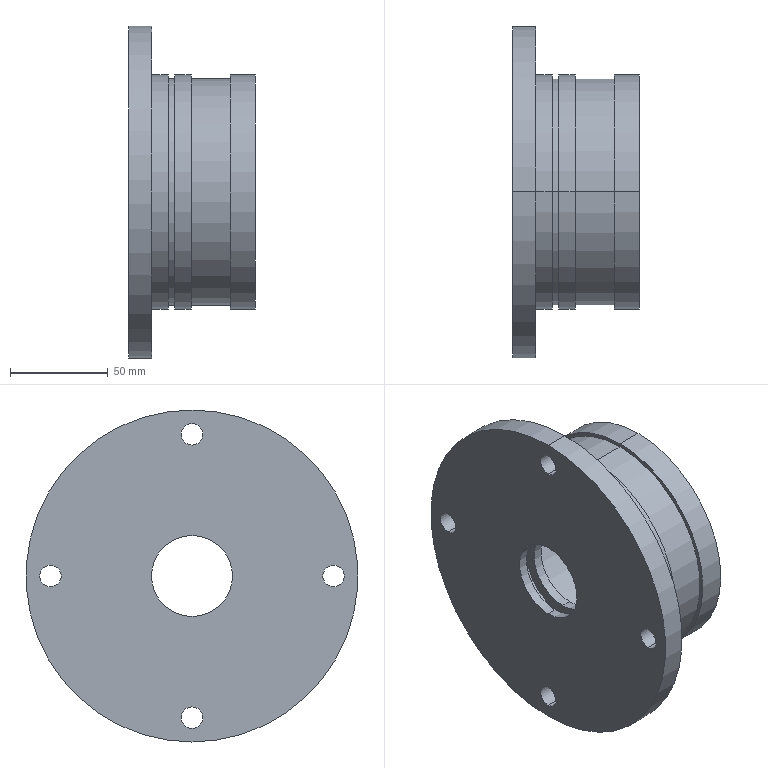Component | SolidWorks | 3FrontCover-1 | 1 solid | 44 faces | box 65 x 170 x 170 mm | volume 391032 mm3 | cylinder 32 | plane 12 | commonest cylinder face diameters 11 x8 120 x6 41.5 x4 116 x4 53 x2 70 x2 100 x2 104 x2
build123d program:
from build123d import *

# Parameters (mm, degrees)
SKETCH74_R           = 85
BOSS_EXTRUDE21_DEPTH = 12
SKETCH75_R           = 60
BOSS_EXTRUDE22_DEPTH = 53
CUT_EXTRUDE18_START  = -33
SKETCH76_2_R         = 60
SKETCH76_2_R_2       = 58
CUT_EXTRUDE18_DEPTH  = 20
CUT_EXTRUDE19_START  = -44.775
SKETCH76_2_2_R       = 60
SKETCH76_2_2_R_2     = 58
CUT_EXTRUDE19_DEPTH  = 3.55
BOSS_EXTRUDE23_START = -8
SKETCH80_R           = 35
BOSS_EXTRUDE23_DEPTH = 15.4
SKETCH81_R           = 20.75
CUT_EXTRUDE20_DEPTH  = 5
SKETCH82_R           = 26.5
CUT_EXTRUDE21_DEPTH  = 5.4
SKETCH83_R           = 20.75
CUT_EXTRUDE22_DEPTH  = 5.4
SKETCH84_R           = 5.5
CUT_EXTRUDE23_DEPTH  = 132.374
CIRPATTERN4_COUNT    = 4


with BuildPart() as part:
    # Sketch74 → Boss-Extrude21 (new body)
    with BuildSketch(Plane(origin=(0, 0, 0), x_dir=(0, 0, -1), z_dir=(1, 0, 0))):
        Circle(SKETCH74_R)
    extrude(amount=BOSS_EXTRUDE21_DEPTH)

    # Sketch75 → Boss-Extrude22 (add)
    with BuildSketch(Plane(origin=(12, 0, 0), x_dir=(0, 0, -1), z_dir=(1, 0, 0))):
        Circle(SKETCH75_R)
    extrude(amount=BOSS_EXTRUDE22_DEPTH)

    # Sketch76_2 → Cut-Extrude18 (cut)
    with BuildSketch(Plane(origin=(65, 0, 0), x_dir=(0, 0, -1), z_dir=(1, 0, 0)).offset(CUT_EXTRUDE18_START)):
        Circle(SKETCH76_2_R)
        Circle(SKETCH76_2_R_2, mode=Mode.SUBTRACT)
    extrude(amount=CUT_EXTRUDE18_DEPTH, mode=Mode.SUBTRACT)

    # Sketch76_2 2 → Cut-Extrude19 (cut)
    with BuildSketch(Plane(origin=(65, 0, 0), x_dir=(0, 0, -1), z_dir=(1, 0, 0)).offset(CUT_EXTRUDE19_START)):
        Circle(SKETCH76_2_2_R)
        Circle(SKETCH76_2_2_R_2, mode=Mode.SUBTRACT)
    extrude(amount=CUT_EXTRUDE19_DEPTH, mode=Mode.SUBTRACT)

    # Sketch78 → Cut-Revolve1 (revolve, cut)
    with BuildSketch(Plane.XY, mode=Mode.PRIVATE) as cut_revolve1_sk:
        Polygon((65, 50), (30, 50), (30, 52), (8, 52), (8, 0), (65, 0), align=None)
    revolve(cut_revolve1_sk.sketch.rotate(Axis((-72.213, 0, 0), (1, 0, 0)), 90), axis=Axis((-72.213, 0, 0), (1, 0, 0)), mode=Mode.SUBTRACT)

    # Sketch80 → Boss-Extrude23 (add)
    with BuildSketch(Plane(origin=(8, 0, 0), x_dir=(0, 0, -1), z_dir=(1, 0, 0)).offset(BOSS_EXTRUDE23_START)):
        with Locations(Location((0, 0, 0), (0, 0, 180))):
            Circle(SKETCH80_R)
    extrude(amount=BOSS_EXTRUDE23_DEPTH)

    # Sketch81 → Cut-Extrude20 (cut)
    with BuildSketch(Plane(origin=(15.4, 0, 0), x_dir=(0, 0, -1), z_dir=(1, 0, 0))):
        Circle(SKETCH81_R)
    extrude(amount=-CUT_EXTRUDE20_DEPTH, mode=Mode.SUBTRACT)

    # Sketch82 → Cut-Extrude21 (cut)
    with BuildSketch(Plane(origin=(10.4, 0, 0), x_dir=(0, 0, -1), z_dir=(1, 0, 0))):
        Circle(SKETCH82_R)
    extrude(amount=-CUT_EXTRUDE21_DEPTH, mode=Mode.SUBTRACT)

    # Sketch83 → Cut-Extrude22 (cut)
    with BuildSketch(Plane(origin=(5, 0, 0), x_dir=(0, 0, -1), z_dir=(1, 0, 0))):
        Circle(SKETCH83_R)
    extrude(amount=-CUT_EXTRUDE22_DEPTH, mode=Mode.SUBTRACT)

    # Sketch84 → Cut-Extrude23 (cut, through all)
    with BuildSketch(Plane(origin=(12, 0, 0), x_dir=(0, 0, -1), z_dir=(1, 0, 0))):
        with Locations((0, 72.5)):
            Circle(SKETCH84_R)
    cut_extrude23 = extrude(amount=-CUT_EXTRUDE23_DEPTH, mode=Mode.SUBTRACT)

    # CirPattern4: Cut-Extrude23 ×4 about axis
    cirpattern4_axis = Axis((0, 0, 0), (1, 0, 0))
    for i in range(1, CIRPATTERN4_COUNT):
        add(cut_extrude23.rotate(cirpattern4_axis, i * 360 / CIRPATTERN4_COUNT), mode=Mode.SUBTRACT)


solid = part.part

# Placed as in the assembly
solid = solid.moved(Location((-167.115, -90.191, 512), (0, 0, 0)))